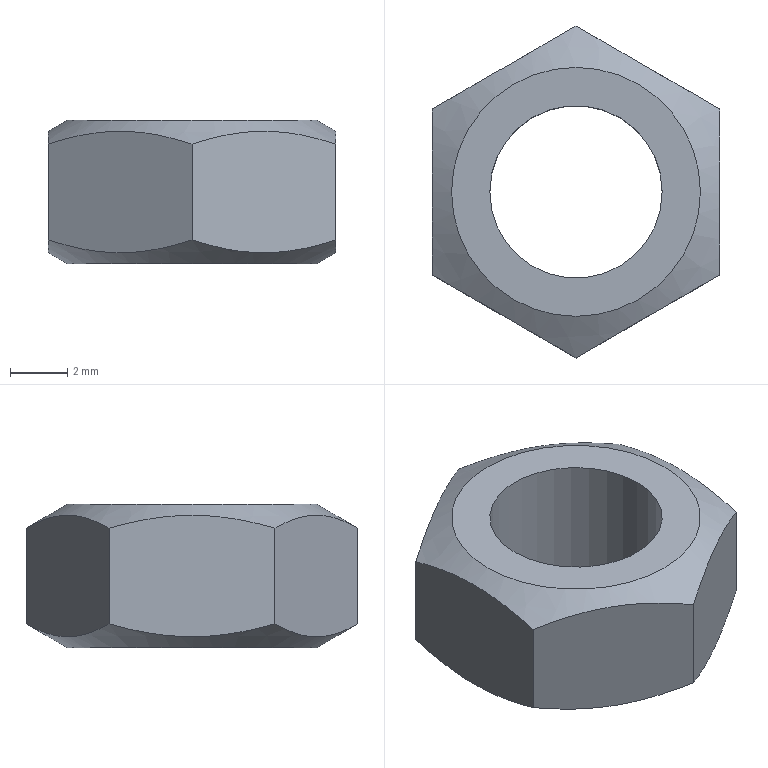Component | NX | NUT | 1 solid | 11 faces | volume 275 mm3 | plane 8 | cone 2 | cylinder 1 | commonest cylinder face diameters 6 x1